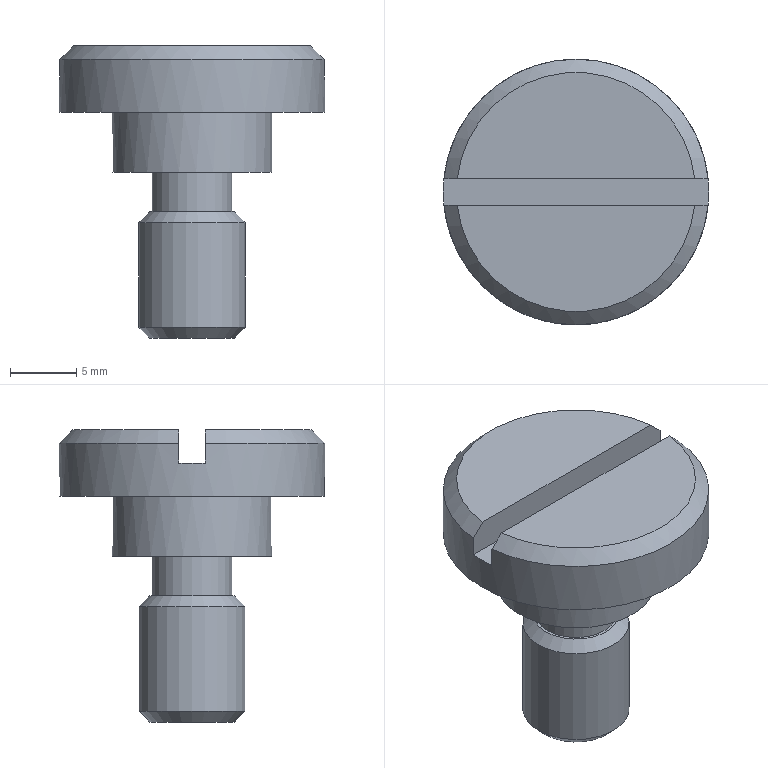Component | NX | DRILL_BUSHING_SCREW | 1 solid | 17 faces | volume 2499 mm3 | plane 9 | cylinder 4 | cone 4 | commonest cylinder face diameters 8 x1 6 x1 12 x1 20 x1